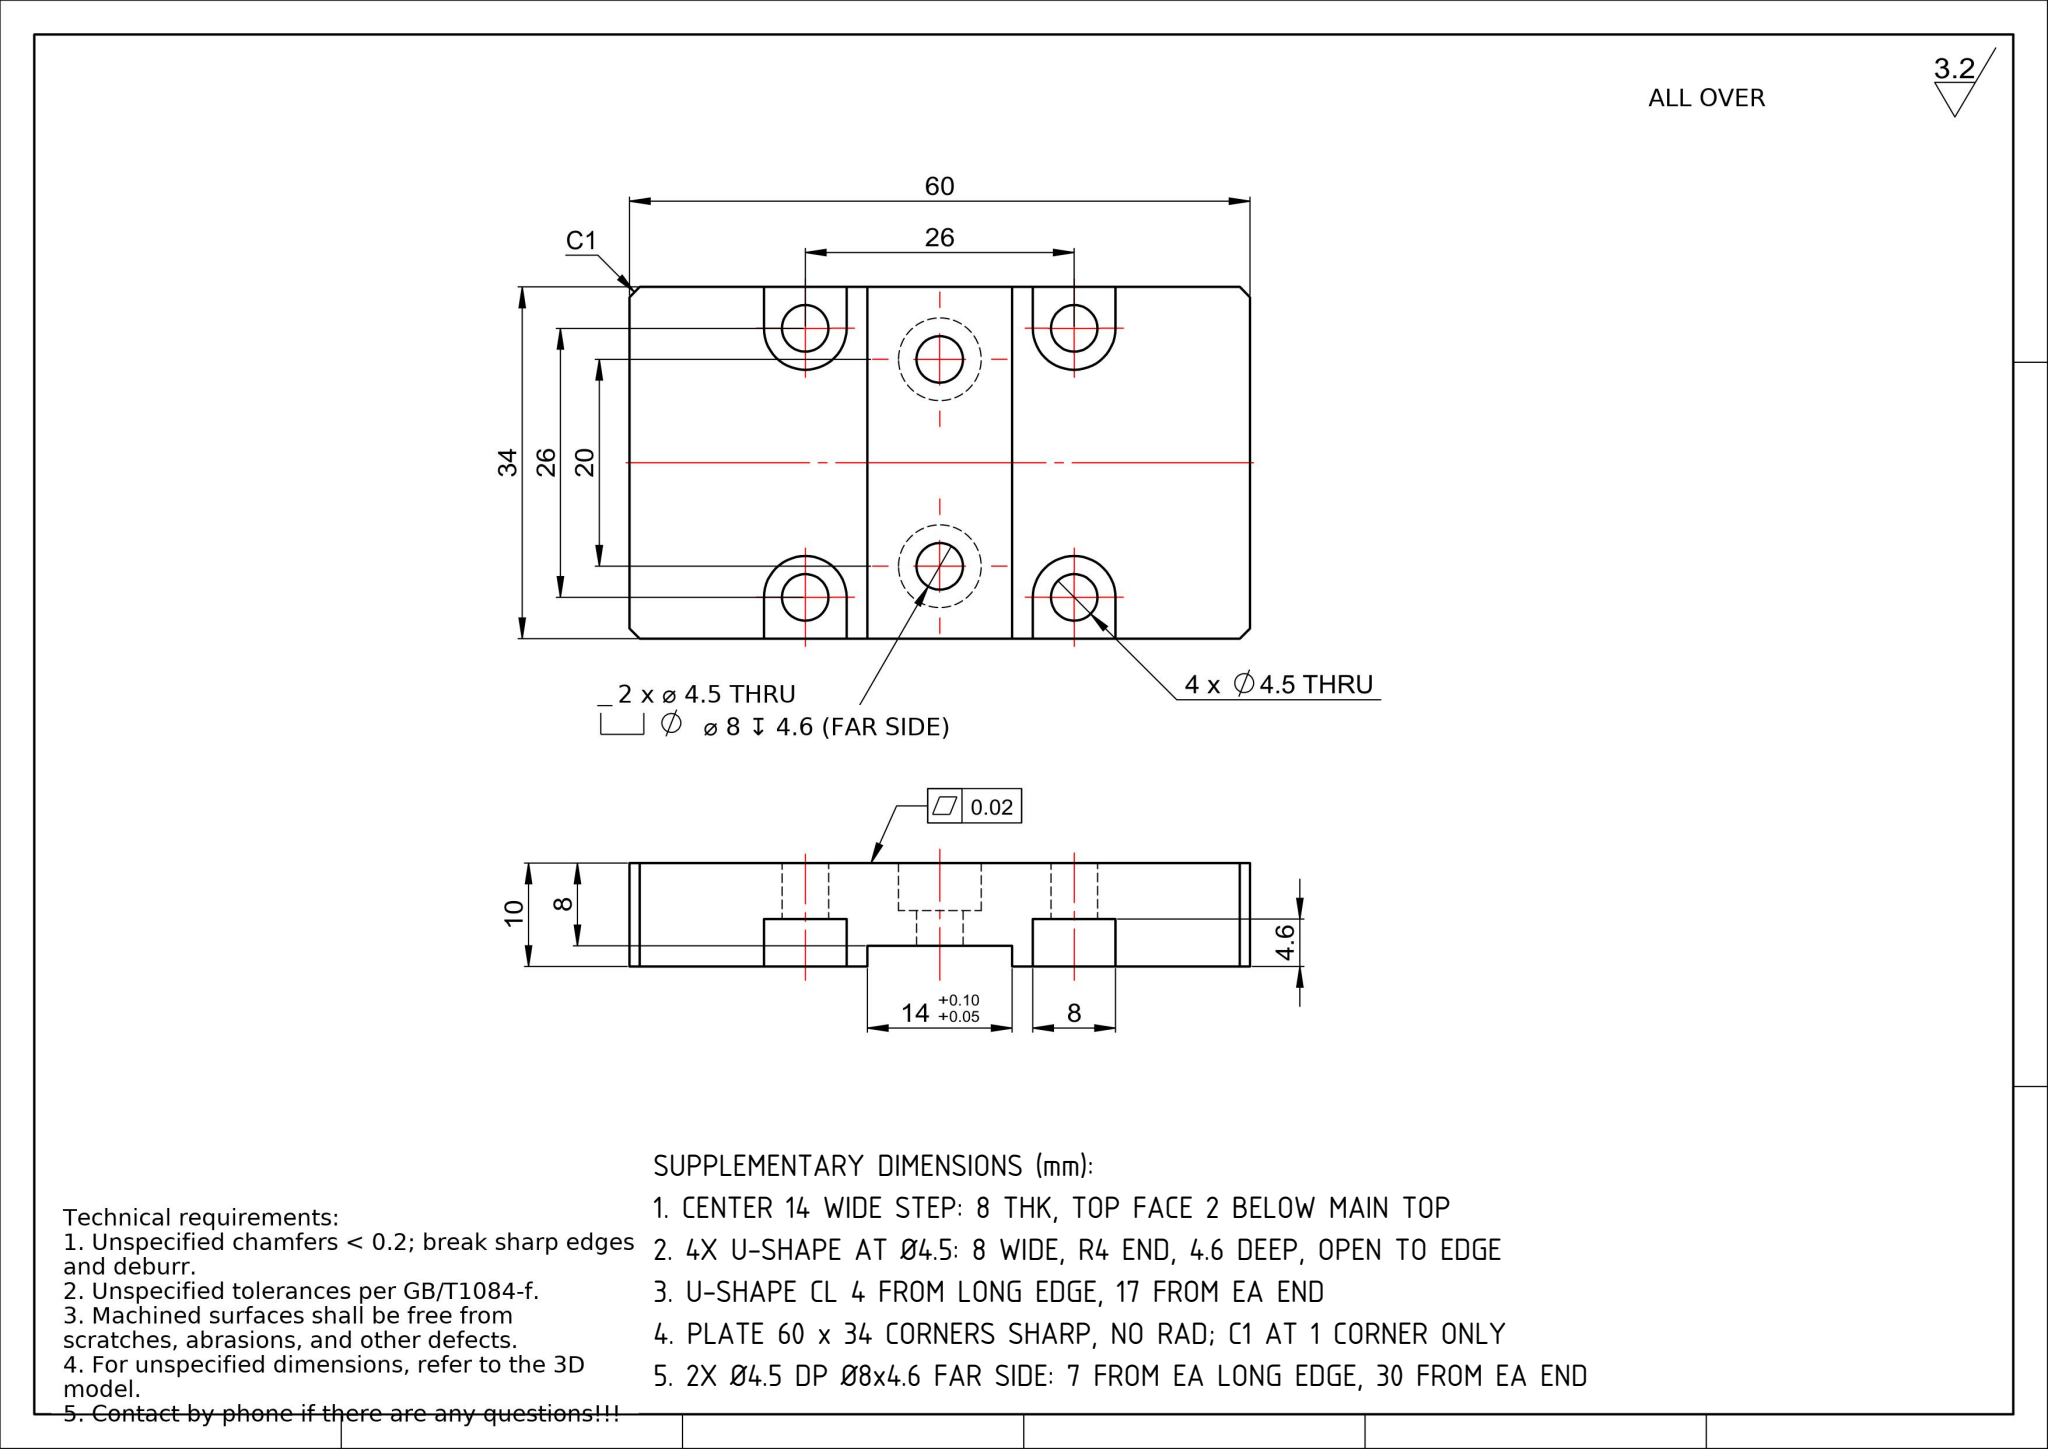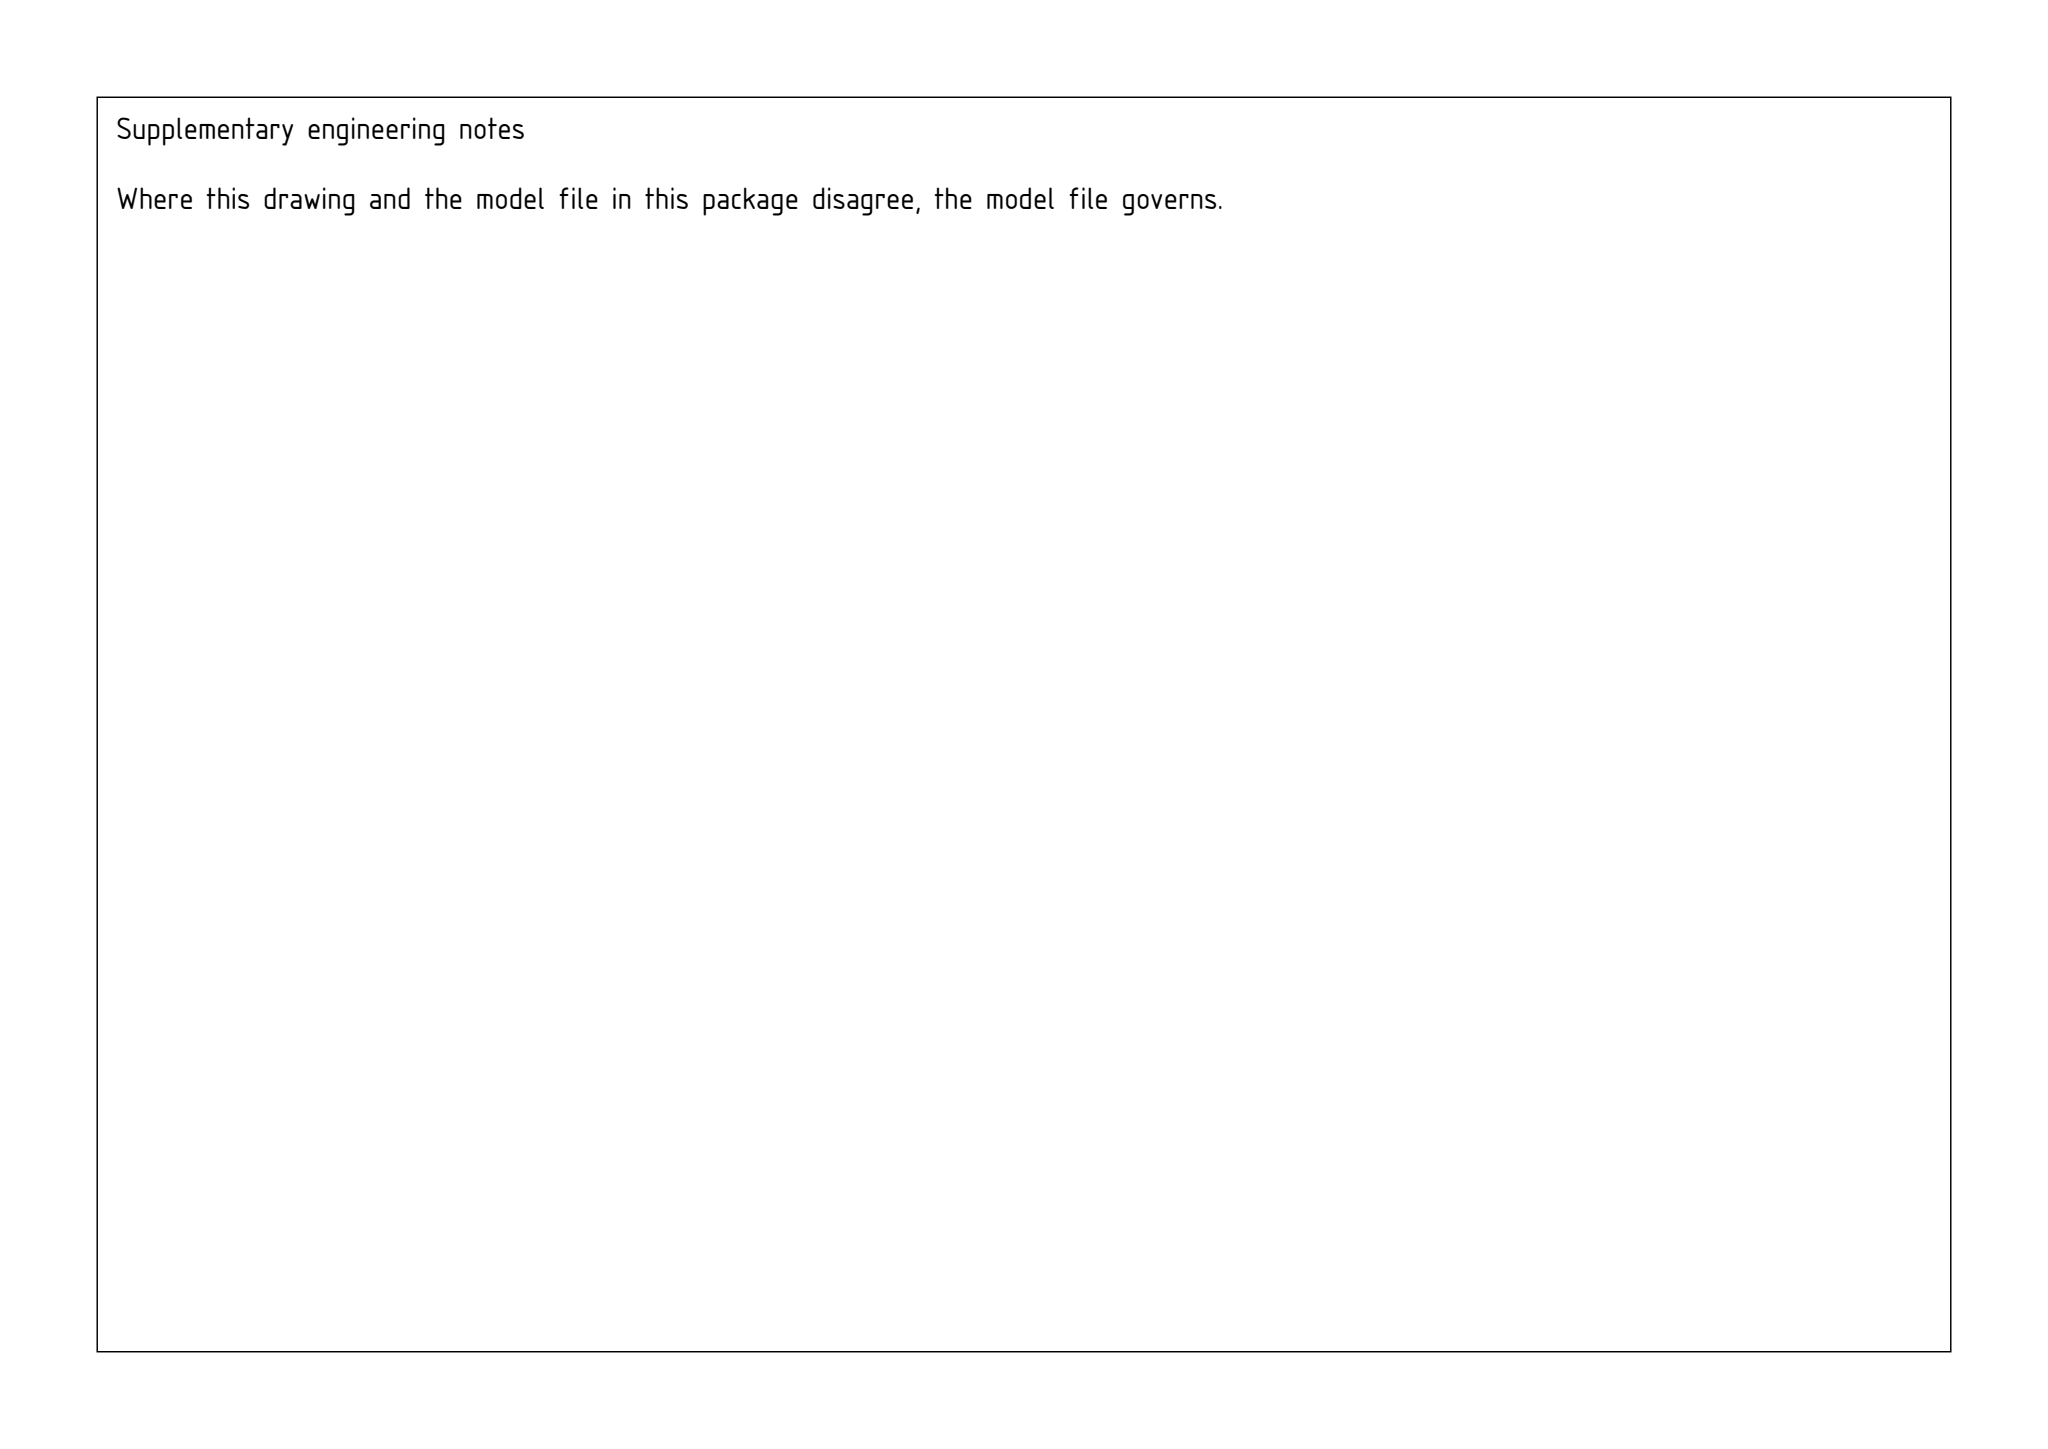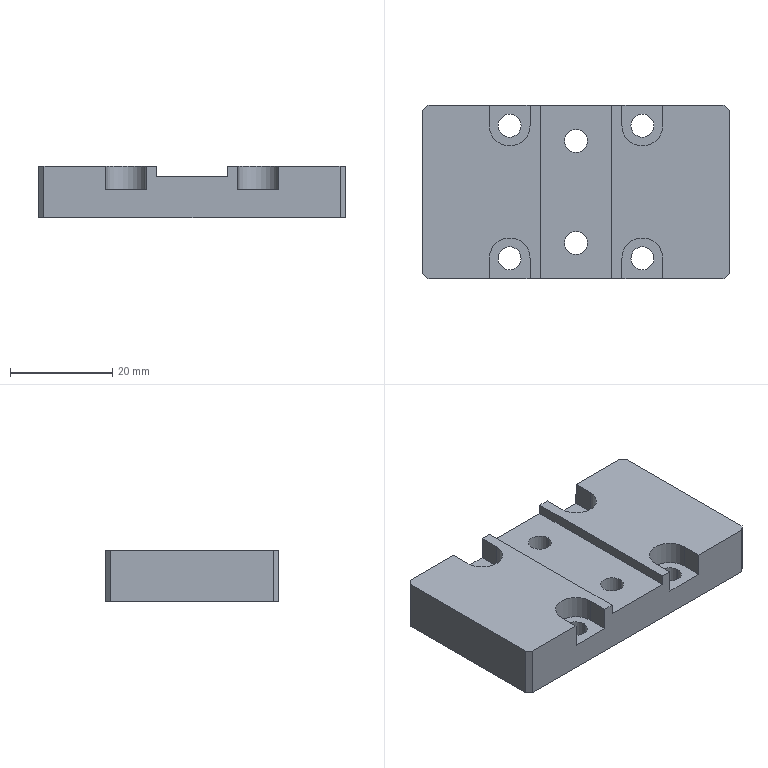Part | SolidWorks | mm | 1 solid | 48 faces | box 60 x 34 x 10 mm | volume 17463 mm3 | plane 28 | cylinder 20 | commonest cylinder face diameters 4.5 x12 8 x8
build123d program:
from build123d import *

# Parameters (mm, degrees)
SKETCH1_W                                            = 60
SKETCH1_H                                            = 34
BOSS_EXTRUDE1_DEPTH                                  = 5
SKETCH2_W                                            = 14
SKETCH2_H                                            = 42.172
CUT_EXTRUDE1_DEPTH                                   = 2
SKETCH5_R                                            = 2.25
CUT_EXTRUDE2_DEPTH                                   = 36.903
CUT_EXTRUDE3_DEPTH                                   = 4.6
HOLE_SIZE_ACCORDING_TO_HEXAGON_SOCKET_HE_D           = 4.5
HOLE_SIZE_ACCORDING_TO_HEXAGON_SOCKET_HE_CBORE_D     = 8
HOLE_SIZE_ACCORDING_TO_HEXAGON_SOCKET_HE_CBORE_DEPTH = 4.6
CHAMFER1_SIZE                                        = 1


with BuildPart() as part:
    # Sketch1 → Boss-Extrude1 (new, symmetric)
    with BuildSketch(Plane.XY):
        Rectangle(SKETCH1_W, SKETCH1_H)
    extrude(amount=BOSS_EXTRUDE1_DEPTH, both=True)

    # Sketch2 → Cut-Extrude1 (cut)
    with BuildSketch(Plane.XY.offset(5)):
        Rectangle(SKETCH2_W, SKETCH2_H)
    extrude(amount=-CUT_EXTRUDE1_DEPTH, mode=Mode.SUBTRACT)

    # Sketch5 → Cut-Extrude2 (cut, through all)
    with BuildSketch(Plane.XY.offset(5)):
        with Locations((-13, 13)):
            Circle(SKETCH5_R)
        with Locations((-13, -13)):
            Circle(SKETCH5_R)
        with Locations((13, 13)):
            Circle(SKETCH5_R)
        with Locations((13, -13)):
            Circle(SKETCH5_R)
    extrude(amount=-CUT_EXTRUDE2_DEPTH, mode=Mode.SUBTRACT)

    # Sketch6 → Cut-Extrude3 (cut)
    with BuildSketch(Plane.XY.offset(5)):
        with BuildLine():
            Line((-17, 13), (-17, 19.725))
            ThreePointArc((-17, 19.725), (-13, 23.725), (-9, 19.725))
            Line((-9, 19.725), (-9, 13))
            ThreePointArc((-9, 13), (-13, 9), (-17, 13))
        make_face()
        with BuildLine():
            Line((9, 13), (9, 19.725))
            ThreePointArc((9, 19.725), (13, 23.725), (17, 19.725))
            Line((17, 19.725), (17, 13))
            ThreePointArc((17, 13), (13, 9), (9, 13))
        make_face()
        with BuildLine():
            Line((-9, -13), (-9, -19.725))
            ThreePointArc((-9, -19.725), (-13, -23.725), (-17, -19.725))
            Line((-17, -19.725), (-17, -13))
            ThreePointArc((-17, -13), (-13, -9), (-9, -13))
        make_face()
        with BuildLine():
            Line((17, -13), (17, -19.725))
            ThreePointArc((17, -19.725), (13, -23.725), (9, -19.725))
            Line((9, -19.725), (9, -13))
            ThreePointArc((9, -13), (13, -9), (17, -13))
        make_face()
    extrude(amount=-CUT_EXTRUDE3_DEPTH, mode=Mode.SUBTRACT)

    # Hole Size according to Hexagon Socket He (through all)
    with Locations(Plane(origin=(0, 0, -5), x_dir=(-1, 0, 0), z_dir=(0, 0, -1))):
        with Locations((0, -10), (0, 10)):
            CounterBoreHole(HOLE_SIZE_ACCORDING_TO_HEXAGON_SOCKET_HE_D / 2, HOLE_SIZE_ACCORDING_TO_HEXAGON_SOCKET_HE_CBORE_D / 2, HOLE_SIZE_ACCORDING_TO_HEXAGON_SOCKET_HE_CBORE_DEPTH)

    # Chamfer1
    chamfer1_edges = [part.edges().sort_by_distance(p)[0] for p in [
        (30, -17, 0),
        (-30, -17, 0),
        (-30, 17, 0),
        (30, 17, 0),
    ]]
    chamfer(chamfer1_edges, length=CHAMFER1_SIZE)


solid = part.part